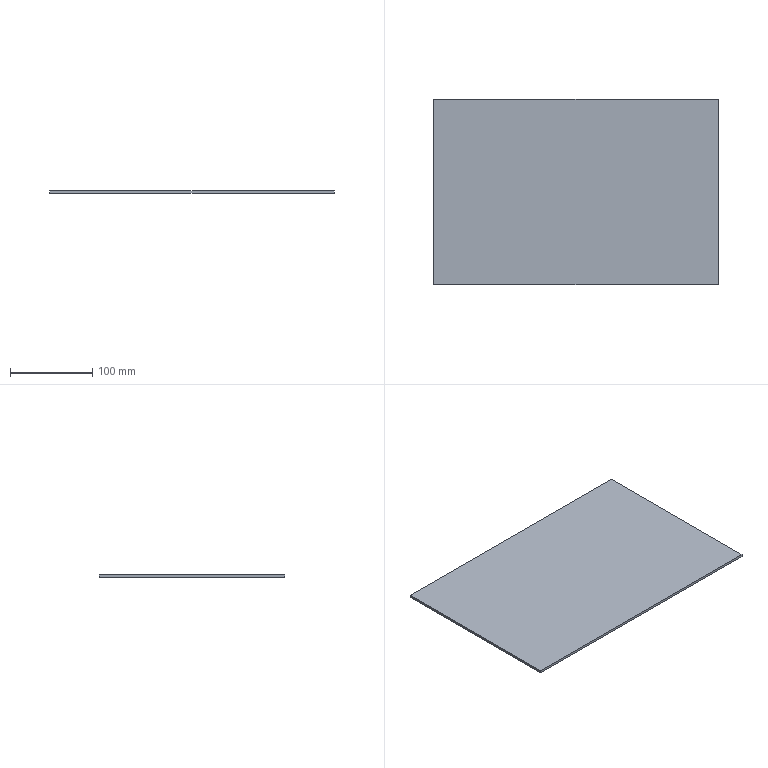Component | SolidWorks | AD12-huiiuban.SDPRT-1 | 1 solid | 6 faces | box 346 x 225 x 3 mm | volume 233550 mm3 | plane 6
build123d program:
from build123d import *

# Parameters (mm, degrees)
SKETCH1_W           = 346
SKETCH1_H           = 225
BOSS_EXTRUDE1_DEPTH = 3


with BuildPart() as part:
    # Sketch1 → Boss-Extrude1 (new body)
    with BuildSketch(Plane.XY):
        Rectangle(SKETCH1_W, SKETCH1_H)
    extrude(amount=BOSS_EXTRUDE1_DEPTH)


solid = part.part

# Placed as in the assembly
solid = solid.moved(Location((-191.414, -16.461, 329.12), (0, 0, 0)))
STEP:
#1=COLOUR_RGB('',0.7922,0.8196,0.9333);
#2=FILL_AREA_STYLE_COLOUR('',#1);
#3=FILL_AREA_STYLE('',(#2));
#4=SURFACE_STYLE_FILL_AREA(#3);
#5=SURFACE_SIDE_STYLE('',(#4));
#6=SURFACE_STYLE_USAGE(.BOTH.,#5);
#7=PRESENTATION_STYLE_ASSIGNMENT((#6));
#8=CARTESIAN_POINT('',(-14.347,3.781,12.957));
#9=VERTEX_POINT('',#8);
#10=CARTESIAN_POINT('',(-14.347,-5.077,12.957));
#11=VERTEX_POINT('',#10);
#12=CARTESIAN_POINT('',(-14.347,-5.077,12.957));
#13=DIRECTION('',(0.,-1.,0.));
#14=VECTOR('',#13,39.37);
#15=LINE('',#12,#14);
#16=EDGE_CURVE('',#9,#11,#15,.T.);
#17=ORIENTED_EDGE('',*,*,#16,.T.);
#18=CARTESIAN_POINT('',(-14.347,-5.077,13.076));
#19=VERTEX_POINT('',#18);
#20=CARTESIAN_POINT('',(-14.347,-5.077,13.076));
#21=DIRECTION('',(0.,0.,-1.));
#22=VECTOR('',#21,39.37);
#23=LINE('',#20,#22);
#24=EDGE_CURVE('',#19,#11,#23,.T.);
#25=ORIENTED_EDGE('',*,*,#24,.F.);
#26=CARTESIAN_POINT('',(-14.347,3.781,13.076));
#27=VERTEX_POINT('',#26);
#28=CARTESIAN_POINT('',(-14.347,-5.077,13.076));
#29=DIRECTION('',(0.,-1.,0.));
#30=VECTOR('',#29,39.37);
#31=LINE('',#28,#30);
#32=EDGE_CURVE('',#27,#19,#31,.T.);
#33=ORIENTED_EDGE('',*,*,#32,.F.);
#34=CARTESIAN_POINT('',(-14.347,3.781,13.076));
#35=DIRECTION('',(0.,0.,-1.));
#36=VECTOR('',#35,39.37);
#37=LINE('',#34,#36);
#38=EDGE_CURVE('',#27,#9,#37,.T.);
#39=ORIENTED_EDGE('',*,*,#38,.T.);
#40=EDGE_LOOP('',(#17,#25,#33,#39));
#41=FACE_OUTER_BOUND('',#40,.T.);
#42=CARTESIAN_POINT('',(-14.347,-5.077,13.076));
#43=DIRECTION('',(1.,0.,0.));
#44=DIRECTION('',(0.,0.,-1.));
#45=AXIS2_PLACEMENT_3D('',#42,#43,#44);
#46=PLANE('',#45);
#47=ADVANCED_FACE('',(#41),#46,.F.);
#48=CARTESIAN_POINT('',(-0.725,-5.077,12.957));
#49=VERTEX_POINT('',#48);
#50=CARTESIAN_POINT('',(-0.725,-5.077,12.957));
#51=DIRECTION('',(1.,0.,0.));
#52=VECTOR('',#51,39.37);
#53=LINE('',#50,#52);
#54=EDGE_CURVE('',#11,#49,#53,.T.);
#55=ORIENTED_EDGE('',*,*,#54,.T.);
#56=CARTESIAN_POINT('',(-0.725,-5.077,13.076));
#57=VERTEX_POINT('',#56);
#58=CARTESIAN_POINT('',(-0.725,-5.077,13.076));
#59=DIRECTION('',(0.,0.,-1.));
#60=VECTOR('',#59,39.37);
#61=LINE('',#58,#60);
#62=EDGE_CURVE('',#57,#49,#61,.T.);
#63=ORIENTED_EDGE('',*,*,#62,.F.);
#64=CARTESIAN_POINT('',(-0.725,-5.077,13.076));
#65=DIRECTION('',(1.,0.,0.));
#66=VECTOR('',#65,39.37);
#67=LINE('',#64,#66);
#68=EDGE_CURVE('',#19,#57,#67,.T.);
#69=ORIENTED_EDGE('',*,*,#68,.F.);
#70=ORIENTED_EDGE('',*,*,#24,.T.);
#71=EDGE_LOOP('',(#55,#63,#69,#70));
#72=FACE_OUTER_BOUND('',#71,.T.);
#73=CARTESIAN_POINT('',(-0.725,-5.077,13.076));
#74=DIRECTION('',(-0.,1.,0.));
#75=DIRECTION('',(-1.,-0.,0.));
#76=AXIS2_PLACEMENT_3D('',#73,#74,#75);
#77=PLANE('',#76);
#78=ADVANCED_FACE('',(#72),#77,.F.);
#79=CARTESIAN_POINT('',(-0.725,3.781,12.957));
#80=VERTEX_POINT('',#79);
#81=CARTESIAN_POINT('',(-0.725,-5.077,12.957));
#82=DIRECTION('',(0.,1.,0.));
#83=VECTOR('',#82,39.37);
#84=LINE('',#81,#83);
#85=EDGE_CURVE('',#49,#80,#84,.T.);
#86=ORIENTED_EDGE('',*,*,#85,.T.);
#87=CARTESIAN_POINT('',(-0.725,3.781,13.076));
#88=VERTEX_POINT('',#87);
#89=CARTESIAN_POINT('',(-0.725,3.781,13.076));
#90=DIRECTION('',(0.,0.,-1.));
#91=VECTOR('',#90,39.37);
#92=LINE('',#89,#91);
#93=EDGE_CURVE('',#88,#80,#92,.T.);
#94=ORIENTED_EDGE('',*,*,#93,.F.);
#95=CARTESIAN_POINT('',(-0.725,-5.077,13.076));
#96=DIRECTION('',(0.,1.,0.));
#97=VECTOR('',#96,39.37);
#98=LINE('',#95,#97);
#99=EDGE_CURVE('',#57,#88,#98,.T.);
#100=ORIENTED_EDGE('',*,*,#99,.F.);
#101=ORIENTED_EDGE('',*,*,#62,.T.);
#102=EDGE_LOOP('',(#86,#94,#100,#101));
#103=FACE_OUTER_BOUND('',#102,.T.);
#104=CARTESIAN_POINT('',(-0.725,-5.077,13.076));
#105=DIRECTION('',(-1.,0.,0.));
#106=DIRECTION('',(0.,0.,1.));
#107=AXIS2_PLACEMENT_3D('',#104,#105,#106);
#108=PLANE('',#107);
#109=ADVANCED_FACE('',(#103),#108,.F.);
#110=CARTESIAN_POINT('',(-0.725,3.781,12.957));
#111=DIRECTION('',(-1.,-0.,0.));
#112=VECTOR('',#111,39.37);
#113=LINE('',#110,#112);
#114=EDGE_CURVE('',#80,#9,#113,.T.);
#115=ORIENTED_EDGE('',*,*,#114,.T.);
#116=ORIENTED_EDGE('',*,*,#38,.F.);
#117=CARTESIAN_POINT('',(-0.725,3.781,13.076));
#118=DIRECTION('',(-1.,-0.,0.));
#119=VECTOR('',#118,39.37);
#120=LINE('',#117,#119);
#121=EDGE_CURVE('',#88,#27,#120,.T.);
#122=ORIENTED_EDGE('',*,*,#121,.F.);
#123=ORIENTED_EDGE('',*,*,#93,.T.);
#124=EDGE_LOOP('',(#115,#116,#122,#123));
#125=FACE_OUTER_BOUND('',#124,.T.);
#126=CARTESIAN_POINT('',(-0.725,3.781,13.076));
#127=DIRECTION('',(0.,-1.,0.));
#128=DIRECTION('',(1.,0.,0.));
#129=AXIS2_PLACEMENT_3D('',#126,#127,#128);
#130=PLANE('',#129);
#131=ADVANCED_FACE('',(#125),#130,.F.);
#132=ORIENTED_EDGE('',*,*,#32,.T.);
#133=ORIENTED_EDGE('',*,*,#68,.T.);
#134=ORIENTED_EDGE('',*,*,#99,.T.);
#135=ORIENTED_EDGE('',*,*,#121,.T.);
#136=EDGE_LOOP('',(#132,#133,#134,#135));
#137=FACE_OUTER_BOUND('',#136,.T.);
#138=CARTESIAN_POINT('',(-7.536,-0.6481,13.076));
#139=DIRECTION('',(0.,0.,1.));
#140=DIRECTION('',(1.,0.,0.));
#141=AXIS2_PLACEMENT_3D('',#138,#139,#140);
#142=PLANE('',#141);
#143=ADVANCED_FACE('',(#137),#142,.T.);
#144=ORIENTED_EDGE('',*,*,#16,.F.);
#145=ORIENTED_EDGE('',*,*,#114,.F.);
#146=ORIENTED_EDGE('',*,*,#85,.F.);
#147=ORIENTED_EDGE('',*,*,#54,.F.);
#148=EDGE_LOOP('',(#144,#145,#146,#147));
#149=FACE_OUTER_BOUND('',#148,.T.);
#150=CARTESIAN_POINT('',(-7.536,-0.6481,12.957));
#151=DIRECTION('',(0.,0.,1.));
#152=DIRECTION('',(1.,0.,0.));
#153=AXIS2_PLACEMENT_3D('',#150,#151,#152);
#154=PLANE('',#153);
#155=ADVANCED_FACE('',(#149),#154,.F.);
#156=CLOSED_SHELL('',(#47,#78,#109,#131,#143,#155));
#157=MANIFOLD_SOLID_BREP('',#156);
#158=STYLED_ITEM('',(#7),#157);
#159=(LENGTH_UNIT()NAMED_UNIT(*)SI_UNIT($,.METRE.));
#160=LENGTH_MEASURE_WITH_UNIT(LENGTH_MEASURE(0.0254),#159);
#161=DIMENSIONAL_EXPONENTS(1.,0.,0.,0.,0.,0.,0.);
#162=(CONVERSION_BASED_UNIT('',#160)LENGTH_UNIT()NAMED_UNIT(#161));
#163=UNCERTAINTY_MEASURE_WITH_UNIT(LENGTH_MEASURE(0.00001),#162,'','');
#164=(NAMED_UNIT(*)PLANE_ANGLE_UNIT()SI_UNIT($,.RADIAN.));
#165=(NAMED_UNIT(*)SI_UNIT($,.STERADIAN.)SOLID_ANGLE_UNIT());
#166=(GEOMETRIC_REPRESENTATION_CONTEXT(3)GLOBAL_UNCERTAINTY_ASSIGNED_CONTEXT((#163))GLOBAL_UNIT_ASSIGNED_CONTEXT((#162,#164,#165))REPRESENTATION_CONTEXT('',''));
#167=MECHANICAL_DESIGN_GEOMETRIC_PRESENTATION_REPRESENTATION('',(#158),#166);
#168=PRESENTATION_LAYER_ASSIGNMENT('','',(#158));
#169=CARTESIAN_POINT('',(0.,0.,0.));
#170=DIRECTION('',(0.,0.,1.));
#171=DIRECTION('',(1.,0.,0.));
#172=AXIS2_PLACEMENT_3D('',#169,#170,#171);
#173=(LENGTH_UNIT()NAMED_UNIT(*)SI_UNIT($,.METRE.));
#174=LENGTH_MEASURE_WITH_UNIT(LENGTH_MEASURE(0.0254),#173);
#175=DIMENSIONAL_EXPONENTS(1.,0.,0.,0.,0.,0.,0.);
#176=(CONVERSION_BASED_UNIT('',#174)LENGTH_UNIT()NAMED_UNIT(#175));
#177=UNCERTAINTY_MEASURE_WITH_UNIT(LENGTH_MEASURE(0.00001),#176,'','');
#178=(NAMED_UNIT(*)PLANE_ANGLE_UNIT()SI_UNIT($,.RADIAN.));
#179=(NAMED_UNIT(*)SI_UNIT($,.STERADIAN.)SOLID_ANGLE_UNIT());
#180=(GEOMETRIC_REPRESENTATION_CONTEXT(3)GLOBAL_UNCERTAINTY_ASSIGNED_CONTEXT((#177))GLOBAL_UNIT_ASSIGNED_CONTEXT((#176,#178,#179))REPRESENTATION_CONTEXT('',''));
#181=ADVANCED_BREP_SHAPE_REPRESENTATION('',(#157,#172),#180);